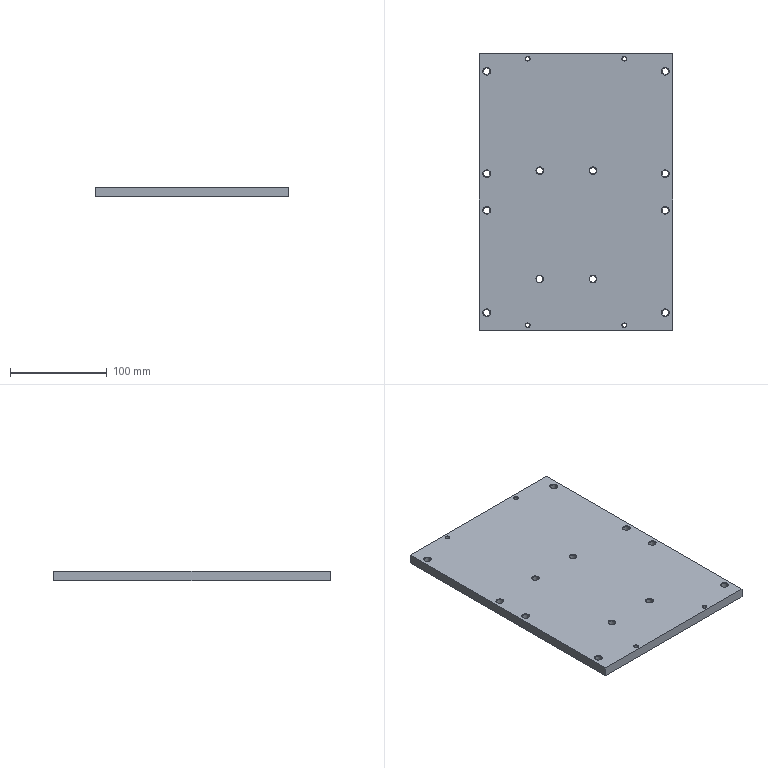Component | NX | FIXED_PLATE_12 | 1 solid | 54 faces | volume 566981 mm3 | cone 32 | cylinder 16 | plane 6 | commonest cylinder face diameters 6.8 x12 4.2 x4